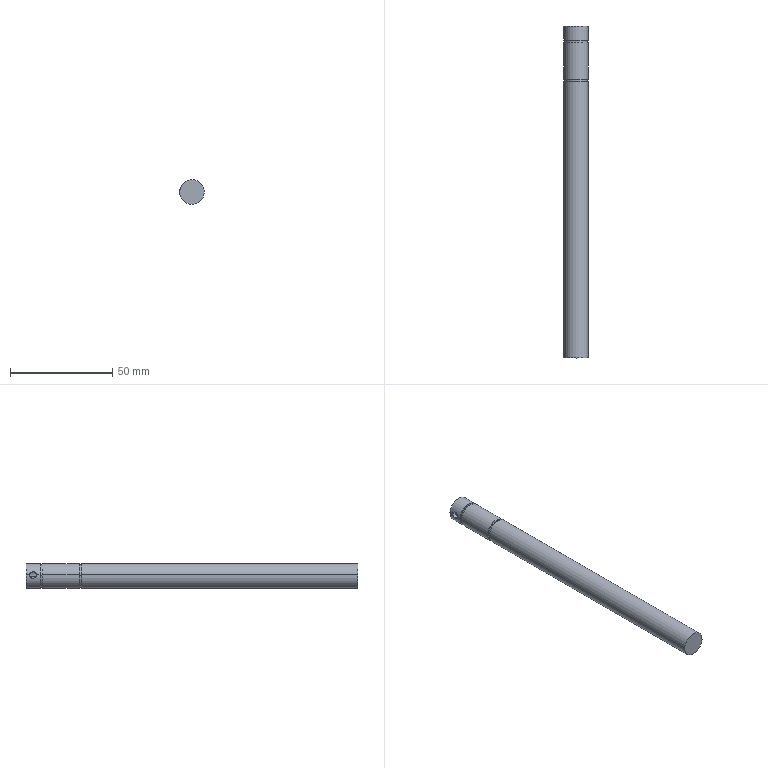Component | SolidWorks | MotorAxis-1 | 1 solid | 21 faces | box 12 x 162 x 12 mm | volume 16498 mm3 | cylinder 14 | plane 7 | commonest cylinder face diameters 12 x6 10.8 x4 3.3 x2 8 x2
build123d program:
from build123d import *

# Parameters (mm, degrees)
SKETCH1_R              = 6
BOSS_EXTRUDE1_DEPTH    = 162
SKETCH2_R              = 4
CUT_EXTRUDE1_DEPTH     = 35
SKETCH3_W              = 4.532
SKETCH3_H              = 1.1
SKETCH3_W_2            = 5.035
M4_TAPPED_HOLE1_REACH  = 161.164
M4_TAPPED_HOLE1_BORE_R = 1.65


with BuildPart() as part:
    # Sketch1 → Boss-Extrude1 (new body)
    with BuildSketch(Plane.XY):
        Circle(SKETCH1_R)
    extrude(amount=BOSS_EXTRUDE1_DEPTH)

    # Sketch2 → Cut-Extrude1 (cut)
    with BuildSketch(Plane(origin=(0, 0, 0), x_dir=(-1, 0, 0), z_dir=(0, 0, -1))):
        Circle(SKETCH2_R)
    extrude(amount=-CUT_EXTRUDE1_DEPTH, mode=Mode.SUBTRACT)

    # Sketch3 → Cut-Revolve1 (revolve, cut)
    with BuildSketch(Plane(origin=(0, 0, 0), x_dir=(1, 0, 0), z_dir=(0, 1, 0)), mode=Mode.PRIVATE) as cut_revolve1_sk:
        with Locations((7.666, -7.45)):
            Rectangle(SKETCH3_W, SKETCH3_H)
        with Locations((7.918, -26.55)):
            Rectangle(SKETCH3_W_2, SKETCH3_H)
    revolve(cut_revolve1_sk.sketch.rotate(Axis((0, 0, 0), (0, 0, 1)), 180), axis=Axis((0, 0, 0), (0, 0, 1)), mode=Mode.SUBTRACT)

    # M4 Tapped Hole1 bore (on position points) → M4 Tapped Hole1 (cut, up to next)
    with BuildSketch(Plane(origin=(-6, 0, 3.403), x_dir=(0, 0, -1), z_dir=(-1, 0, 0)), mode=Mode.PRIVATE) as m4_tapped_hole1_sk1:
        Circle(M4_TAPPED_HOLE1_BORE_R)
    m4_tapped_hole1_tool1 = extrude(m4_tapped_hole1_sk1.sketch, amount=-M4_TAPPED_HOLE1_REACH, mode=Mode.PRIVATE) & part.part
    add(m4_tapped_hole1_tool1.solids().sort_by_distance((-6, 0, 3.403))[0], mode=Mode.SUBTRACT)


solid = part.part

# Placed as in the assembly
solid = solid.moved(Location((-48.547, 4.46, 328), (90, 0, -5.004)))
STEP:
#1=COLOUR_RGB('',0.7922,0.8196,0.9333);
#2=FILL_AREA_STYLE_COLOUR('',#1);
#3=FILL_AREA_STYLE('',(#2));
#4=SURFACE_STYLE_FILL_AREA(#3);
#5=SURFACE_SIDE_STYLE('',(#4));
#6=SURFACE_STYLE_USAGE(.BOTH.,#5);
#7=PRESENTATION_STYLE_ASSIGNMENT((#6));
#8=CARTESIAN_POINT('',(-2.068,0.1066,12.927));
#9=VERTEX_POINT('',#8);
#10=CARTESIAN_POINT('',(-2.068,-0.02332,12.927));
#11=VERTEX_POINT('',#10);
#12=CARTESIAN_POINT('',(-2.068,0.1066,12.927));
#13=CARTESIAN_POINT('',(-2.069,0.1066,12.923));
#14=CARTESIAN_POINT('',(-2.069,0.1062,12.919));
#15=CARTESIAN_POINT('',(-2.069,0.1045,12.91));
#16=CARTESIAN_POINT('',(-2.069,0.1032,12.906));
#17=CARTESIAN_POINT('',(-2.068,0.0983,12.894));
#18=CARTESIAN_POINT('',(-2.067,0.09352,12.887));
#19=CARTESIAN_POINT('',(-2.065,0.08454,12.878));
#20=CARTESIAN_POINT('',(-2.064,0.0813,12.875));
#21=CARTESIAN_POINT('',(-2.063,0.07433,12.87));
#22=CARTESIAN_POINT('',(-2.062,0.07055,12.868));
#23=CARTESIAN_POINT('',(-2.061,0.06272,12.865));
#24=CARTESIAN_POINT('',(-2.061,0.05867,12.863));
#25=CARTESIAN_POINT('',(-2.06,0.05029,12.862));
#26=CARTESIAN_POINT('',(-2.06,0.04593,12.861));
#27=CARTESIAN_POINT('',(-2.06,0.03309,12.861));
#28=CARTESIAN_POINT('',(-2.061,0.02447,12.863));
#29=CARTESIAN_POINT('',(-2.062,0.01273,12.868));
#30=CARTESIAN_POINT('',(-2.063,0.008947,12.87));
#31=CARTESIAN_POINT('',(-2.064,0.001949,12.875));
#32=CARTESIAN_POINT('',(-2.065,-0.001288,12.878));
#33=CARTESIAN_POINT('',(-2.066,-0.007255,12.884));
#34=CARTESIAN_POINT('',(-2.067,-0.009956,12.887));
#35=CARTESIAN_POINT('',(-2.068,-0.01464,12.894));
#36=CARTESIAN_POINT('',(-2.068,-0.01664,12.898));
#37=CARTESIAN_POINT('',(-2.069,-0.02161,12.91));
#38=CARTESIAN_POINT('',(-2.069,-0.02332,12.918));
#39=CARTESIAN_POINT('',(-2.068,-0.02332,12.927));
#40=B_SPLINE_CURVE_WITH_KNOTS('',3,(#12,#13,#14,#15,#16,#17,#18,#19,#20,#21,#22,#23,#24,#25,#26,#27,#28,#29,#30,#31,#32,#33,#34,#35,#36,#37,#38,#39),.UNSPECIFIED.,.F.,.F.,(4,2,2,2,2,2,2,2,2,2,2,2,2,4),(0.005218,0.005543,0.005869,0.006521,0.006847,0.007173,0.007499,0.007824,0.008476,0.008802,0.009128,0.009454,0.009779,0.01043),.UNSPECIFIED.);
#41=EDGE_CURVE('',#9,#11,#40,.T.);
#42=ORIENTED_EDGE('',*,*,#41,.F.);
#43=CARTESIAN_POINT('',(-2.147,0.1066,12.934));
#44=VERTEX_POINT('',#43);
#45=CARTESIAN_POINT('',(-2.147,0.1066,12.934));
#46=DIRECTION('',(-0.9962,-0.,0.08723));
#47=VECTOR('',#46,39.37);
#48=LINE('',#45,#47);
#49=EDGE_CURVE('',#9,#44,#48,.T.);
#50=ORIENTED_EDGE('',*,*,#49,.T.);
#51=CARTESIAN_POINT('',(-2.147,-0.02332,12.934));
#52=VERTEX_POINT('',#51);
#53=CARTESIAN_POINT('',(-2.147,-0.02332,12.934));
#54=CARTESIAN_POINT('',(-2.147,-0.02332,12.93));
#55=CARTESIAN_POINT('',(-2.147,-0.0229,12.925));
#56=CARTESIAN_POINT('',(-2.148,-0.02123,12.917));
#57=CARTESIAN_POINT('',(-2.148,-0.01997,12.913));
#58=CARTESIAN_POINT('',(-2.147,-0.0167,12.905));
#59=CARTESIAN_POINT('',(-2.147,-0.01471,12.901));
#60=CARTESIAN_POINT('',(-2.147,-0.009991,12.894));
#61=CARTESIAN_POINT('',(-2.146,-0.007262,12.891));
#62=CARTESIAN_POINT('',(-2.145,0.001683,12.882));
#63=CARTESIAN_POINT('',(-2.145,0.008896,12.877));
#64=CARTESIAN_POINT('',(-2.144,0.02451,12.87));
#65=CARTESIAN_POINT('',(-2.143,0.03309,12.868));
#66=CARTESIAN_POINT('',(-2.143,0.04587,12.868));
#67=CARTESIAN_POINT('',(-2.143,0.0502,12.869));
#68=CARTESIAN_POINT('',(-2.144,0.05855,12.871));
#69=CARTESIAN_POINT('',(-2.144,0.06261,12.872));
#70=CARTESIAN_POINT('',(-2.145,0.07444,12.877));
#71=CARTESIAN_POINT('',(-2.145,0.08158,12.882));
#72=CARTESIAN_POINT('',(-2.146,0.09059,12.891));
#73=CARTESIAN_POINT('',(-2.147,0.09326,12.894));
#74=CARTESIAN_POINT('',(-2.147,0.09796,12.901));
#75=CARTESIAN_POINT('',(-2.147,0.1,12.905));
#76=CARTESIAN_POINT('',(-2.148,0.1033,12.913));
#77=CARTESIAN_POINT('',(-2.148,0.1045,12.917));
#78=CARTESIAN_POINT('',(-2.147,0.1062,12.925));
#79=CARTESIAN_POINT('',(-2.147,0.1066,12.93));
#80=CARTESIAN_POINT('',(-2.147,0.1066,12.934));
#81=B_SPLINE_CURVE_WITH_KNOTS('',3,(#53,#54,#55,#56,#57,#58,#59,#60,#61,#62,#63,#64,#65,#66,#67,#68,#69,#70,#71,#72,#73,#74,#75,#76,#77,#78,#79,#80),.UNSPECIFIED.,.F.,.F.,(4,2,2,2,2,2,2,2,2,2,2,2,2,4),(0.,0.000324,0.000648,0.000972,0.001296,0.001944,0.002592,0.002916,0.00324,0.003888,0.004212,0.004536,0.00486,0.005184),.UNSPECIFIED.);
#82=EDGE_CURVE('',#52,#44,#81,.T.);
#83=ORIENTED_EDGE('',*,*,#82,.F.);
#84=CARTESIAN_POINT('',(-2.147,-0.02332,12.934));
#85=DIRECTION('',(-0.9962,-0.,0.08723));
#86=VECTOR('',#85,39.37);
#87=LINE('',#84,#86);
#88=EDGE_CURVE('',#11,#52,#87,.T.);
#89=ORIENTED_EDGE('',*,*,#88,.F.);
#90=EDGE_LOOP('',(#42,#50,#83,#89));
#91=FACE_OUTER_BOUND('',#90,.T.);
#92=CARTESIAN_POINT('',(-2.147,0.04164,12.934));
#93=DIRECTION('',(-0.9962,-0.,0.08723));
#94=DIRECTION('',(0.,-1.,0.));
#95=AXIS2_PLACEMENT_3D('',#92,#93,#94);
#96=CYLINDRICAL_SURFACE('',#95,0.06496);
#97=ADVANCED_FACE('',(#91),#96,.F.);
#98=CARTESIAN_POINT('',(-1.676,-6.202,12.893));
#99=VERTEX_POINT('',#98);
#100=CARTESIAN_POINT('',(-2.147,-6.202,12.934));
#101=VERTEX_POINT('',#100);
#102=CARTESIAN_POINT('',(-1.911,-6.202,12.913));
#103=DIRECTION('',(0.,-1.,0.));
#104=DIRECTION('',(0.9962,0.,-0.08723));
#105=AXIS2_PLACEMENT_3D('',#102,#103,#104);
#106=CIRCLE('',#105,0.2362);
#107=EDGE_CURVE('',#99,#101,#106,.T.);
#108=ORIENTED_EDGE('',*,*,#107,.F.);
#109=CARTESIAN_POINT('',(-1.676,-0.8913,12.893));
#110=VERTEX_POINT('',#109);
#111=CARTESIAN_POINT('',(-1.676,-6.202,12.893));
#112=DIRECTION('',(-0.,1.,-0.));
#113=VECTOR('',#112,39.37);
#114=LINE('',#111,#113);
#115=EDGE_CURVE('',#99,#110,#114,.T.);
#116=ORIENTED_EDGE('',*,*,#115,.T.);
#117=CARTESIAN_POINT('',(-2.147,-0.8913,12.934));
#118=VERTEX_POINT('',#117);
#119=CARTESIAN_POINT('',(-1.911,-0.8913,12.913));
#120=DIRECTION('',(-0.,1.,-0.));
#121=DIRECTION('',(-0.9962,-0.,0.08723));
#122=AXIS2_PLACEMENT_3D('',#119,#120,#121);
#123=CIRCLE('',#122,0.2362);
#124=EDGE_CURVE('',#118,#110,#123,.T.);
#125=ORIENTED_EDGE('',*,*,#124,.F.);
#126=CARTESIAN_POINT('',(-2.147,-6.202,12.934));
#127=DIRECTION('',(-0.,1.,-0.));
#128=VECTOR('',#127,39.37);
#129=LINE('',#126,#128);
#130=EDGE_CURVE('',#101,#118,#129,.T.);
#131=ORIENTED_EDGE('',*,*,#130,.F.);
#132=EDGE_LOOP('',(#108,#116,#125,#131));
#133=FACE_OUTER_BOUND('',#132,.T.);
#134=CARTESIAN_POINT('',(-1.911,-6.202,12.913));
#135=DIRECTION('',(-0.,1.,-0.));
#136=DIRECTION('',(-0.9962,0.,0.08723));
#137=AXIS2_PLACEMENT_3D('',#134,#135,#136);
#138=CYLINDRICAL_SURFACE('',#137,0.2362);
#139=ADVANCED_FACE('',(#133),#138,.T.);
#140=CARTESIAN_POINT('',(-2.123,-0.8913,12.932));
#141=VERTEX_POINT('',#140);
#142=CARTESIAN_POINT('',(-1.7,-0.8913,12.895));
#143=VERTEX_POINT('',#142);
#144=CARTESIAN_POINT('',(-1.911,-0.8913,12.913));
#145=DIRECTION('',(-0.,1.,-0.));
#146=DIRECTION('',(-0.9962,-0.,0.08723));
#147=AXIS2_PLACEMENT_3D('',#144,#145,#146);
#148=CIRCLE('',#147,0.2126);
#149=EDGE_CURVE('',#141,#143,#148,.T.);
#150=ORIENTED_EDGE('',*,*,#149,.T.);
#151=CARTESIAN_POINT('',(-1.7,-0.848,12.895));
#152=VERTEX_POINT('',#151);
#153=CARTESIAN_POINT('',(-1.7,0.1756,12.895));
#154=DIRECTION('',(-0.,1.,-0.));
#155=VECTOR('',#154,39.37);
#156=LINE('',#153,#155);
#157=EDGE_CURVE('',#143,#152,#156,.T.);
#158=ORIENTED_EDGE('',*,*,#157,.T.);
#159=CARTESIAN_POINT('',(-2.123,-0.848,12.932));
#160=VERTEX_POINT('',#159);
#161=CARTESIAN_POINT('',(-1.911,-0.848,12.913));
#162=DIRECTION('',(-0.,1.,-0.));
#163=DIRECTION('',(-0.9962,-0.,0.08723));
#164=AXIS2_PLACEMENT_3D('',#161,#162,#163);
#165=CIRCLE('',#164,0.2126);
#166=EDGE_CURVE('',#160,#152,#165,.T.);
#167=ORIENTED_EDGE('',*,*,#166,.F.);
#168=CARTESIAN_POINT('',(-2.123,0.1756,12.932));
#169=DIRECTION('',(-0.,1.,-0.));
#170=VECTOR('',#169,39.37);
#171=LINE('',#168,#170);
#172=EDGE_CURVE('',#141,#160,#171,.T.);
#173=ORIENTED_EDGE('',*,*,#172,.F.);
#174=EDGE_LOOP('',(#150,#158,#167,#173));
#175=FACE_OUTER_BOUND('',#174,.T.);
#176=CARTESIAN_POINT('',(-1.911,0.1756,12.913));
#177=DIRECTION('',(-0.,1.,-0.));
#178=DIRECTION('',(-0.9962,-0.,0.08723));
#179=AXIS2_PLACEMENT_3D('',#176,#177,#178);
#180=CYLINDRICAL_SURFACE('',#179,0.2126);
#181=ADVANCED_FACE('',(#175),#180,.T.);
#182=CARTESIAN_POINT('',(-2.123,-0.1394,12.932));
#183=VERTEX_POINT('',#182);
#184=CARTESIAN_POINT('',(-1.7,-0.1394,12.895));
#185=VERTEX_POINT('',#184);
#186=CARTESIAN_POINT('',(-1.911,-0.1394,12.913));
#187=DIRECTION('',(-0.,1.,-0.));
#188=DIRECTION('',(-0.9962,-0.,0.08723));
#189=AXIS2_PLACEMENT_3D('',#186,#187,#188);
#190=CIRCLE('',#189,0.2126);
#191=EDGE_CURVE('',#183,#185,#190,.T.);
#192=ORIENTED_EDGE('',*,*,#191,.T.);
#193=CARTESIAN_POINT('',(-1.7,-0.09605,12.895));
#194=VERTEX_POINT('',#193);
#195=CARTESIAN_POINT('',(-1.7,0.1756,12.895));
#196=DIRECTION('',(-0.,1.,-0.));
#197=VECTOR('',#196,39.37);
#198=LINE('',#195,#197);
#199=EDGE_CURVE('',#185,#194,#198,.T.);
#200=ORIENTED_EDGE('',*,*,#199,.T.);
#201=CARTESIAN_POINT('',(-2.123,-0.09605,12.932));
#202=VERTEX_POINT('',#201);
#203=CARTESIAN_POINT('',(-1.911,-0.09605,12.913));
#204=DIRECTION('',(-0.,1.,-0.));
#205=DIRECTION('',(-0.9962,-0.,0.08723));
#206=AXIS2_PLACEMENT_3D('',#203,#204,#205);
#207=CIRCLE('',#206,0.2126);
#208=EDGE_CURVE('',#202,#194,#207,.T.);
#209=ORIENTED_EDGE('',*,*,#208,.F.);
#210=CARTESIAN_POINT('',(-2.123,0.1756,12.932));
#211=DIRECTION('',(-0.,1.,-0.));
#212=VECTOR('',#211,39.37);
#213=LINE('',#210,#212);
#214=EDGE_CURVE('',#183,#202,#213,.T.);
#215=ORIENTED_EDGE('',*,*,#214,.F.);
#216=EDGE_LOOP('',(#192,#200,#209,#215));
#217=FACE_OUTER_BOUND('',#216,.T.);
#218=CARTESIAN_POINT('',(-1.911,0.1756,12.913));
#219=DIRECTION('',(-0.,1.,-0.));
#220=DIRECTION('',(-0.9962,-0.,0.08723));
#221=AXIS2_PLACEMENT_3D('',#218,#219,#220);
#222=CYLINDRICAL_SURFACE('',#221,0.2126);
#223=ADVANCED_FACE('',(#217),#222,.T.);
#224=CARTESIAN_POINT('',(-1.754,-1.202,12.9));
#225=VERTEX_POINT('',#224);
#226=CARTESIAN_POINT('',(-2.068,-1.202,12.927));
#227=VERTEX_POINT('',#226);
#228=CARTESIAN_POINT('',(-1.911,-1.202,12.913));
#229=DIRECTION('',(-0.,1.,-0.));
#230=DIRECTION('',(-0.9962,-0.,0.08723));
#231=AXIS2_PLACEMENT_3D('',#228,#229,#230);
#232=CIRCLE('',#231,0.1575);
#233=EDGE_CURVE('',#225,#227,#232,.T.);
#234=ORIENTED_EDGE('',*,*,#233,.F.);
#235=CARTESIAN_POINT('',(-1.754,0.1756,12.9));
#236=VERTEX_POINT('',#235);
#237=CARTESIAN_POINT('',(-1.754,-1.202,12.9));
#238=DIRECTION('',(-0.,1.,-0.));
#239=VECTOR('',#238,39.37);
#240=LINE('',#237,#239);
#241=EDGE_CURVE('',#225,#236,#240,.T.);
#242=ORIENTED_EDGE('',*,*,#241,.T.);
#243=CARTESIAN_POINT('',(-2.068,0.1756,12.927));
#244=VERTEX_POINT('',#243);
#245=CARTESIAN_POINT('',(-1.911,0.1756,12.913));
#246=DIRECTION('',(-0.,1.,-0.));
#247=DIRECTION('',(-0.9962,-0.,0.08723));
#248=AXIS2_PLACEMENT_3D('',#245,#246,#247);
#249=CIRCLE('',#248,0.1575);
#250=EDGE_CURVE('',#236,#244,#249,.T.);
#251=ORIENTED_EDGE('',*,*,#250,.T.);
#252=CARTESIAN_POINT('',(-2.068,-1.202,12.927));
#253=DIRECTION('',(-0.,1.,-0.));
#254=VECTOR('',#253,39.37);
#255=LINE('',#252,#254);
#256=EDGE_CURVE('',#9,#244,#255,.T.);
#257=ORIENTED_EDGE('',*,*,#256,.F.);
#258=ORIENTED_EDGE('',*,*,#41,.T.);
#259=CARTESIAN_POINT('',(-2.068,-1.202,12.927));
#260=DIRECTION('',(-0.,1.,-0.));
#261=VECTOR('',#260,39.37);
#262=LINE('',#259,#261);
#263=EDGE_CURVE('',#227,#11,#262,.T.);
#264=ORIENTED_EDGE('',*,*,#263,.F.);
#265=EDGE_LOOP('',(#234,#242,#251,#257,#258,#264));
#266=FACE_OUTER_BOUND('',#265,.T.);
#267=CARTESIAN_POINT('',(-1.911,-1.202,12.913));
#268=DIRECTION('',(-0.,1.,-0.));
#269=DIRECTION('',(-0.9962,-0.,0.08723));
#270=AXIS2_PLACEMENT_3D('',#267,#268,#269);
#271=CYLINDRICAL_SURFACE('',#270,0.1575);
#272=ADVANCED_FACE('',(#266),#271,.F.);
#273=CARTESIAN_POINT('',(-1.676,-0.09605,12.893));
#274=VERTEX_POINT('',#273);
#275=CARTESIAN_POINT('',(-2.147,-0.09605,12.934));
#276=VERTEX_POINT('',#275);
#277=CARTESIAN_POINT('',(-1.911,-0.09605,12.913));
#278=DIRECTION('',(0.,-1.,0.));
#279=DIRECTION('',(0.9962,0.,-0.08723));
#280=AXIS2_PLACEMENT_3D('',#277,#278,#279);
#281=CIRCLE('',#280,0.2362);
#282=EDGE_CURVE('',#274,#276,#281,.T.);
#283=ORIENTED_EDGE('',*,*,#282,.F.);
#284=CARTESIAN_POINT('',(-1.676,0.1756,12.893));
#285=VERTEX_POINT('',#284);
#286=CARTESIAN_POINT('',(-1.676,-6.202,12.893));
#287=DIRECTION('',(-0.,1.,-0.));
#288=VECTOR('',#287,39.37);
#289=LINE('',#286,#288);
#290=EDGE_CURVE('',#274,#285,#289,.T.);
#291=ORIENTED_EDGE('',*,*,#290,.T.);
#292=CARTESIAN_POINT('',(-2.147,0.1756,12.934));
#293=VERTEX_POINT('',#292);
#294=CARTESIAN_POINT('',(-1.911,0.1756,12.913));
#295=DIRECTION('',(0.,-1.,0.));
#296=DIRECTION('',(0.9962,0.,-0.08723));
#297=AXIS2_PLACEMENT_3D('',#294,#295,#296);
#298=CIRCLE('',#297,0.2362);
#299=EDGE_CURVE('',#285,#293,#298,.T.);
#300=ORIENTED_EDGE('',*,*,#299,.T.);
#301=CARTESIAN_POINT('',(-2.147,-6.202,12.934));
#302=DIRECTION('',(-0.,1.,-0.));
#303=VECTOR('',#302,39.37);
#304=LINE('',#301,#303);
#305=EDGE_CURVE('',#44,#293,#304,.T.);
#306=ORIENTED_EDGE('',*,*,#305,.F.);
#307=CARTESIAN_POINT('',(-2.147,0.1066,12.934));
#308=CARTESIAN_POINT('',(-2.146,0.1066,12.942));
#309=CARTESIAN_POINT('',(-2.145,0.1049,12.951));
#310=CARTESIAN_POINT('',(-2.142,0.1,12.963));
#311=CARTESIAN_POINT('',(-2.142,0.09797,12.966));
#312=CARTESIAN_POINT('',(-2.14,0.09325,12.973));
#313=CARTESIAN_POINT('',(-2.139,0.09058,12.976));
#314=CARTESIAN_POINT('',(-2.137,0.08459,12.982));
#315=CARTESIAN_POINT('',(-2.136,0.08127,12.985));
#316=CARTESIAN_POINT('',(-2.135,0.07427,12.99));
#317=CARTESIAN_POINT('',(-2.134,0.07054,12.991));
#318=CARTESIAN_POINT('',(-2.133,0.06263,12.995));
#319=CARTESIAN_POINT('',(-2.133,0.05856,12.996));
#320=CARTESIAN_POINT('',(-2.132,0.05024,12.997));
#321=CARTESIAN_POINT('',(-2.132,0.04593,12.998));
#322=CARTESIAN_POINT('',(-2.132,0.03737,12.998));
#323=CARTESIAN_POINT('',(-2.132,0.03314,12.998));
#324=CARTESIAN_POINT('',(-2.133,0.02478,12.996));
#325=CARTESIAN_POINT('',(-2.133,0.02064,12.995));
#326=CARTESIAN_POINT('',(-2.135,0.008894,12.99));
#327=CARTESIAN_POINT('',(-2.136,0.001688,12.985));
#328=CARTESIAN_POINT('',(-2.14,-0.01023,12.974));
#329=CARTESIAN_POINT('',(-2.142,-0.01507,12.966));
#330=CARTESIAN_POINT('',(-2.144,-0.01996,12.955));
#331=CARTESIAN_POINT('',(-2.145,-0.02122,12.951));
#332=CARTESIAN_POINT('',(-2.146,-0.0229,12.943));
#333=CARTESIAN_POINT('',(-2.146,-0.02332,12.938));
#334=CARTESIAN_POINT('',(-2.147,-0.02332,12.934));
#335=B_SPLINE_CURVE_WITH_KNOTS('',3,(#307,#308,#309,#310,#311,#312,#313,#314,#315,#316,#317,#318,#319,#320,#321,#322,#323,#324,#325,#326,#327,#328,#329,#330,#331,#332,#333,#334),.UNSPECIFIED.,.F.,.F.,(4,2,2,2,2,2,2,2,2,2,2,2,2,4),(0.005184,0.005832,0.006155,0.006479,0.006803,0.007127,0.007451,0.007775,0.008099,0.008423,0.00907,0.009718,0.01004,0.01037),.UNSPECIFIED.);
#336=EDGE_CURVE('',#44,#52,#335,.T.);
#337=ORIENTED_EDGE('',*,*,#336,.T.);
#338=CARTESIAN_POINT('',(-2.147,-6.202,12.934));
#339=DIRECTION('',(-0.,1.,-0.));
#340=VECTOR('',#339,39.37);
#341=LINE('',#338,#340);
#342=EDGE_CURVE('',#276,#52,#341,.T.);
#343=ORIENTED_EDGE('',*,*,#342,.F.);
#344=EDGE_LOOP('',(#283,#291,#300,#306,#337,#343));
#345=FACE_OUTER_BOUND('',#344,.T.);
#346=CARTESIAN_POINT('',(-1.911,-6.202,12.913));
#347=DIRECTION('',(-0.,1.,-0.));
#348=DIRECTION('',(-0.9962,0.,0.08723));
#349=AXIS2_PLACEMENT_3D('',#346,#347,#348);
#350=CYLINDRICAL_SURFACE('',#349,0.2362);
#351=ADVANCED_FACE('',(#345),#350,.T.);
#352=CARTESIAN_POINT('',(-1.676,-0.848,12.893));
#353=VERTEX_POINT('',#352);
#354=CARTESIAN_POINT('',(-2.147,-0.848,12.934));
#355=VERTEX_POINT('',#354);
#356=CARTESIAN_POINT('',(-1.911,-0.848,12.913));
#357=DIRECTION('',(0.,-1.,0.));
#358=DIRECTION('',(0.9962,0.,-0.08723));
#359=AXIS2_PLACEMENT_3D('',#356,#357,#358);
#360=CIRCLE('',#359,0.2362);
#361=EDGE_CURVE('',#353,#355,#360,.T.);
#362=ORIENTED_EDGE('',*,*,#361,.F.);
#363=CARTESIAN_POINT('',(-1.676,-0.1394,12.893));
#364=VERTEX_POINT('',#363);
#365=CARTESIAN_POINT('',(-1.676,-6.202,12.893));
#366=DIRECTION('',(-0.,1.,-0.));
#367=VECTOR('',#366,39.37);
#368=LINE('',#365,#367);
#369=EDGE_CURVE('',#353,#364,#368,.T.);
#370=ORIENTED_EDGE('',*,*,#369,.T.);
#371=CARTESIAN_POINT('',(-2.147,-0.1394,12.934));
#372=VERTEX_POINT('',#371);
#373=CARTESIAN_POINT('',(-1.911,-0.1394,12.913));
#374=DIRECTION('',(-0.,1.,-0.));
#375=DIRECTION('',(-0.9962,-0.,0.08723));
#376=AXIS2_PLACEMENT_3D('',#373,#374,#375);
#377=CIRCLE('',#376,0.2362);
#378=EDGE_CURVE('',#372,#364,#377,.T.);
#379=ORIENTED_EDGE('',*,*,#378,.F.);
#380=CARTESIAN_POINT('',(-2.147,-6.202,12.934));
#381=DIRECTION('',(-0.,1.,-0.));
#382=VECTOR('',#381,39.37);
#383=LINE('',#380,#382);
#384=EDGE_CURVE('',#355,#372,#383,.T.);
#385=ORIENTED_EDGE('',*,*,#384,.F.);
#386=EDGE_LOOP('',(#362,#370,#379,#385));
#387=FACE_OUTER_BOUND('',#386,.T.);
#388=CARTESIAN_POINT('',(-1.911,-6.202,12.913));
#389=DIRECTION('',(-0.,1.,-0.));
#390=DIRECTION('',(-0.9962,0.,0.08723));
#391=AXIS2_PLACEMENT_3D('',#388,#389,#390);
#392=CYLINDRICAL_SURFACE('',#391,0.2362);
#393=ADVANCED_FACE('',(#387),#392,.T.);
#394=ORIENTED_EDGE('',*,*,#369,.F.);
#395=CARTESIAN_POINT('',(-1.911,-0.848,12.913));
#396=DIRECTION('',(0.,-1.,0.));
#397=DIRECTION('',(0.9962,0.,-0.08723));
#398=AXIS2_PLACEMENT_3D('',#395,#396,#397);
#399=CIRCLE('',#398,0.2362);
#400=EDGE_CURVE('',#355,#353,#399,.T.);
#401=ORIENTED_EDGE('',*,*,#400,.F.);
#402=ORIENTED_EDGE('',*,*,#384,.T.);
#403=CARTESIAN_POINT('',(-1.911,-0.1394,12.913));
#404=DIRECTION('',(-0.,1.,-0.));
#405=DIRECTION('',(-0.9962,-0.,0.08723));
#406=AXIS2_PLACEMENT_3D('',#403,#404,#405);
#407=CIRCLE('',#406,0.2362);
#408=EDGE_CURVE('',#364,#372,#407,.T.);
#409=ORIENTED_EDGE('',*,*,#408,.F.);
#410=EDGE_LOOP('',(#394,#401,#402,#409));
#411=FACE_OUTER_BOUND('',#410,.T.);
#412=CARTESIAN_POINT('',(-1.911,-6.202,12.913));
#413=DIRECTION('',(-0.,1.,-0.));
#414=DIRECTION('',(-0.9962,0.,0.08723));
#415=AXIS2_PLACEMENT_3D('',#412,#413,#414);
#416=CYLINDRICAL_SURFACE('',#415,0.2362);
#417=ADVANCED_FACE('',(#411),#416,.T.);
#418=ORIENTED_EDGE('',*,*,#290,.F.);
#419=CARTESIAN_POINT('',(-1.911,-0.09605,12.913));
#420=DIRECTION('',(0.,-1.,0.));
#421=DIRECTION('',(0.9962,0.,-0.08723));
#422=AXIS2_PLACEMENT_3D('',#419,#420,#421);
#423=CIRCLE('',#422,0.2362);
#424=EDGE_CURVE('',#276,#274,#423,.T.);
#425=ORIENTED_EDGE('',*,*,#424,.F.);
#426=ORIENTED_EDGE('',*,*,#342,.T.);
#427=ORIENTED_EDGE('',*,*,#82,.T.);
#428=ORIENTED_EDGE('',*,*,#305,.T.);
#429=CARTESIAN_POINT('',(-1.911,0.1756,12.913));
#430=DIRECTION('',(0.,-1.,0.));
#431=DIRECTION('',(0.9962,0.,-0.08723));
#432=AXIS2_PLACEMENT_3D('',#429,#430,#431);
#433=CIRCLE('',#432,0.2362);
#434=EDGE_CURVE('',#293,#285,#433,.T.);
#435=ORIENTED_EDGE('',*,*,#434,.T.);
#436=EDGE_LOOP('',(#418,#425,#426,#427,#428,#435));
#437=FACE_OUTER_BOUND('',#436,.T.);
#438=CARTESIAN_POINT('',(-1.911,-6.202,12.913));
#439=DIRECTION('',(-0.,1.,-0.));
#440=DIRECTION('',(-0.9962,0.,0.08723));
#441=AXIS2_PLACEMENT_3D('',#438,#439,#440);
#442=CYLINDRICAL_SURFACE('',#441,0.2362);
#443=ADVANCED_FACE('',(#437),#442,.T.);
#444=CARTESIAN_POINT('',(-1.911,0.1756,12.913));
#445=DIRECTION('',(-0.,1.,-0.));
#446=DIRECTION('',(-0.9962,-0.,0.08723));
#447=AXIS2_PLACEMENT_3D('',#444,#445,#446);
#448=CIRCLE('',#447,0.1575);
#449=EDGE_CURVE('',#244,#236,#448,.T.);
#450=ORIENTED_EDGE('',*,*,#449,.F.);
#451=ORIENTED_EDGE('',*,*,#250,.F.);
#452=EDGE_LOOP('',(#450,#451));
#453=FACE_BOUND('',#452,.T.);
#454=ORIENTED_EDGE('',*,*,#434,.F.);
#455=ORIENTED_EDGE('',*,*,#299,.F.);
#456=EDGE_LOOP('',(#454,#455));
#457=FACE_OUTER_BOUND('',#456,.T.);
#458=CARTESIAN_POINT('',(-1.911,0.1756,12.913));
#459=DIRECTION('',(0.,-1.,0.));
#460=DIRECTION('',(0.9962,0.,-0.08723));
#461=AXIS2_PLACEMENT_3D('',#458,#459,#460);
#462=PLANE('',#461);
#463=ADVANCED_FACE('',(#453,#457),#462,.F.);
#464=ORIENTED_EDGE('',*,*,#241,.F.);
#465=CARTESIAN_POINT('',(-1.911,-1.202,12.913));
#466=DIRECTION('',(-0.,1.,-0.));
#467=DIRECTION('',(-0.9962,-0.,0.08723));
#468=AXIS2_PLACEMENT_3D('',#465,#466,#467);
#469=CIRCLE('',#468,0.1575);
#470=EDGE_CURVE('',#227,#225,#469,.T.);
#471=ORIENTED_EDGE('',*,*,#470,.F.);
#472=ORIENTED_EDGE('',*,*,#263,.T.);
#473=CARTESIAN_POINT('',(-2.068,-0.02332,12.927));
#474=CARTESIAN_POINT('',(-2.068,-0.02332,12.931));
#475=CARTESIAN_POINT('',(-2.067,-0.02289,12.936));
#476=CARTESIAN_POINT('',(-2.066,-0.02121,12.944));
#477=CARTESIAN_POINT('',(-2.065,-0.01994,12.948));
#478=CARTESIAN_POINT('',(-2.062,-0.01501,12.96));
#479=CARTESIAN_POINT('',(-2.06,-0.01019,12.967));
#480=CARTESIAN_POINT('',(-2.055,0.001663,12.978));
#481=CARTESIAN_POINT('',(-2.053,0.008817,12.983));
#482=CARTESIAN_POINT('',(-2.05,0.02051,12.987));
#483=CARTESIAN_POINT('',(-2.05,0.02465,12.989));
#484=CARTESIAN_POINT('',(-2.049,0.03306,12.99));
#485=CARTESIAN_POINT('',(-2.049,0.0373,12.991));
#486=CARTESIAN_POINT('',(-2.049,0.04589,12.991));
#487=CARTESIAN_POINT('',(-2.049,0.05025,12.99));
#488=CARTESIAN_POINT('',(-2.05,0.05862,12.989));
#489=CARTESIAN_POINT('',(-2.05,0.06271,12.987));
#490=CARTESIAN_POINT('',(-2.052,0.07062,12.984));
#491=CARTESIAN_POINT('',(-2.053,0.07433,12.982));
#492=CARTESIAN_POINT('',(-2.055,0.08132,12.978));
#493=CARTESIAN_POINT('',(-2.056,0.08462,12.975));
#494=CARTESIAN_POINT('',(-2.059,0.09056,12.969));
#495=CARTESIAN_POINT('',(-2.06,0.09322,12.966));
#496=CARTESIAN_POINT('',(-2.062,0.09793,12.959));
#497=CARTESIAN_POINT('',(-2.063,0.09996,12.956));
#498=CARTESIAN_POINT('',(-2.066,0.1048,12.944));
#499=CARTESIAN_POINT('',(-2.067,0.1066,12.936));
#500=CARTESIAN_POINT('',(-2.068,0.1066,12.927));
#501=B_SPLINE_CURVE_WITH_KNOTS('',3,(#473,#474,#475,#476,#477,#478,#479,#480,#481,#482,#483,#484,#485,#486,#487,#488,#489,#490,#491,#492,#493,#494,#495,#496,#497,#498,#499,#500),.UNSPECIFIED.,.F.,.F.,(4,2,2,2,2,2,2,2,2,2,2,2,2,4),(0.,0.0003261,0.0006522,0.001304,0.001957,0.002283,0.002609,0.002935,0.003261,0.003587,0.003913,0.004239,0.004565,0.005218),.UNSPECIFIED.);
#502=EDGE_CURVE('',#11,#9,#501,.T.);
#503=ORIENTED_EDGE('',*,*,#502,.T.);
#504=ORIENTED_EDGE('',*,*,#256,.T.);
#505=ORIENTED_EDGE('',*,*,#449,.T.);
#506=EDGE_LOOP('',(#464,#471,#472,#503,#504,#505));
#507=FACE_OUTER_BOUND('',#506,.T.);
#508=CARTESIAN_POINT('',(-1.911,-1.202,12.913));
#509=DIRECTION('',(-0.,1.,-0.));
#510=DIRECTION('',(-0.9962,-0.,0.08723));
#511=AXIS2_PLACEMENT_3D('',#508,#509,#510);
#512=CYLINDRICAL_SURFACE('',#511,0.1575);
#513=ADVANCED_FACE('',(#507),#512,.F.);
#514=ORIENTED_EDGE('',*,*,#470,.T.);
#515=ORIENTED_EDGE('',*,*,#233,.T.);
#516=EDGE_LOOP('',(#514,#515));
#517=FACE_OUTER_BOUND('',#516,.T.);
#518=CARTESIAN_POINT('',(-1.911,-1.202,12.913));
#519=DIRECTION('',(-0.,1.,-0.));
#520=DIRECTION('',(-0.9962,-0.,0.08723));
#521=AXIS2_PLACEMENT_3D('',#518,#519,#520);
#522=PLANE('',#521);
#523=ADVANCED_FACE('',(#517),#522,.T.);
#524=ORIENTED_EDGE('',*,*,#191,.F.);
#525=CARTESIAN_POINT('',(-1.911,-0.1394,12.913));
#526=DIRECTION('',(-0.,1.,-0.));
#527=DIRECTION('',(-0.9962,-0.,0.08723));
#528=AXIS2_PLACEMENT_3D('',#525,#526,#527);
#529=CIRCLE('',#528,0.2126);
#530=EDGE_CURVE('',#185,#183,#529,.T.);
#531=ORIENTED_EDGE('',*,*,#530,.F.);
#532=EDGE_LOOP('',(#524,#531));
#533=FACE_BOUND('',#532,.T.);
#534=ORIENTED_EDGE('',*,*,#378,.T.);
#535=ORIENTED_EDGE('',*,*,#408,.T.);
#536=EDGE_LOOP('',(#534,#535));
#537=FACE_OUTER_BOUND('',#536,.T.);
#538=CARTESIAN_POINT('',(-1.7,-0.1394,12.895));
#539=DIRECTION('',(-0.,1.,-0.));
#540=DIRECTION('',(-0.9962,-0.,0.08723));
#541=AXIS2_PLACEMENT_3D('',#538,#539,#540);
#542=PLANE('',#541);
#543=ADVANCED_FACE('',(#533,#537),#542,.T.);
#544=ORIENTED_EDGE('',*,*,#208,.T.);
#545=CARTESIAN_POINT('',(-1.911,-0.09605,12.913));
#546=DIRECTION('',(-0.,1.,-0.));
#547=DIRECTION('',(-0.9962,-0.,0.08723));
#548=AXIS2_PLACEMENT_3D('',#545,#546,#547);
#549=CIRCLE('',#548,0.2126);
#550=EDGE_CURVE('',#194,#202,#549,.T.);
#551=ORIENTED_EDGE('',*,*,#550,.T.);
#552=EDGE_LOOP('',(#544,#551));
#553=FACE_BOUND('',#552,.T.);
#554=ORIENTED_EDGE('',*,*,#424,.T.);
#555=ORIENTED_EDGE('',*,*,#282,.T.);
#556=EDGE_LOOP('',(#554,#555));
#557=FACE_OUTER_BOUND('',#556,.T.);
#558=CARTESIAN_POINT('',(-1.7,-0.09605,12.895));
#559=DIRECTION('',(0.,-1.,0.));
#560=DIRECTION('',(0.9962,0.,-0.08723));
#561=AXIS2_PLACEMENT_3D('',#558,#559,#560);
#562=PLANE('',#561);
#563=ADVANCED_FACE('',(#553,#557),#562,.T.);
#564=ORIENTED_EDGE('',*,*,#199,.F.);
#565=ORIENTED_EDGE('',*,*,#530,.T.);
#566=ORIENTED_EDGE('',*,*,#214,.T.);
#567=ORIENTED_EDGE('',*,*,#550,.F.);
#568=EDGE_LOOP('',(#564,#565,#566,#567));
#569=FACE_OUTER_BOUND('',#568,.T.);
#570=CARTESIAN_POINT('',(-1.911,0.1756,12.913));
#571=DIRECTION('',(-0.,1.,-0.));
#572=DIRECTION('',(-0.9962,-0.,0.08723));
#573=AXIS2_PLACEMENT_3D('',#570,#571,#572);
#574=CYLINDRICAL_SURFACE('',#573,0.2126);
#575=ADVANCED_FACE('',(#569),#574,.T.);
#576=ORIENTED_EDGE('',*,*,#149,.F.);
#577=CARTESIAN_POINT('',(-1.911,-0.8913,12.913));
#578=DIRECTION('',(-0.,1.,-0.));
#579=DIRECTION('',(-0.9962,-0.,0.08723));
#580=AXIS2_PLACEMENT_3D('',#577,#578,#579);
#581=CIRCLE('',#580,0.2126);
#582=EDGE_CURVE('',#143,#141,#581,.T.);
#583=ORIENTED_EDGE('',*,*,#582,.F.);
#584=EDGE_LOOP('',(#576,#583));
#585=FACE_BOUND('',#584,.T.);
#586=ORIENTED_EDGE('',*,*,#124,.T.);
#587=CARTESIAN_POINT('',(-1.911,-0.8913,12.913));
#588=DIRECTION('',(-0.,1.,-0.));
#589=DIRECTION('',(-0.9962,-0.,0.08723));
#590=AXIS2_PLACEMENT_3D('',#587,#588,#589);
#591=CIRCLE('',#590,0.2362);
#592=EDGE_CURVE('',#110,#118,#591,.T.);
#593=ORIENTED_EDGE('',*,*,#592,.T.);
#594=EDGE_LOOP('',(#586,#593));
#595=FACE_OUTER_BOUND('',#594,.T.);
#596=CARTESIAN_POINT('',(-1.7,-0.8913,12.895));
#597=DIRECTION('',(-0.,1.,-0.));
#598=DIRECTION('',(-0.9962,-0.,0.08723));
#599=AXIS2_PLACEMENT_3D('',#596,#597,#598);
#600=PLANE('',#599);
#601=ADVANCED_FACE('',(#585,#595),#600,.T.);
#602=ORIENTED_EDGE('',*,*,#166,.T.);
#603=CARTESIAN_POINT('',(-1.911,-0.848,12.913));
#604=DIRECTION('',(-0.,1.,-0.));
#605=DIRECTION('',(-0.9962,-0.,0.08723));
#606=AXIS2_PLACEMENT_3D('',#603,#604,#605);
#607=CIRCLE('',#606,0.2126);
#608=EDGE_CURVE('',#152,#160,#607,.T.);
#609=ORIENTED_EDGE('',*,*,#608,.T.);
#610=EDGE_LOOP('',(#602,#609));
#611=FACE_BOUND('',#610,.T.);
#612=ORIENTED_EDGE('',*,*,#400,.T.);
#613=ORIENTED_EDGE('',*,*,#361,.T.);
#614=EDGE_LOOP('',(#612,#613));
#615=FACE_OUTER_BOUND('',#614,.T.);
#616=CARTESIAN_POINT('',(-1.7,-0.848,12.895));
#617=DIRECTION('',(0.,-1.,0.));
#618=DIRECTION('',(0.9962,0.,-0.08723));
#619=AXIS2_PLACEMENT_3D('',#616,#617,#618);
#620=PLANE('',#619);
#621=ADVANCED_FACE('',(#611,#615),#620,.T.);
#622=ORIENTED_EDGE('',*,*,#157,.F.);
#623=ORIENTED_EDGE('',*,*,#582,.T.);
#624=ORIENTED_EDGE('',*,*,#172,.T.);
#625=ORIENTED_EDGE('',*,*,#608,.F.);
#626=EDGE_LOOP('',(#622,#623,#624,#625));
#627=FACE_OUTER_BOUND('',#626,.T.);
#628=CARTESIAN_POINT('',(-1.911,0.1756,12.913));
#629=DIRECTION('',(-0.,1.,-0.));
#630=DIRECTION('',(-0.9962,-0.,0.08723));
#631=AXIS2_PLACEMENT_3D('',#628,#629,#630);
#632=CYLINDRICAL_SURFACE('',#631,0.2126);
#633=ADVANCED_FACE('',(#627),#632,.T.);
#634=CARTESIAN_POINT('',(-1.911,-6.202,12.913));
#635=DIRECTION('',(0.,-1.,0.));
#636=DIRECTION('',(0.9962,0.,-0.08723));
#637=AXIS2_PLACEMENT_3D('',#634,#635,#636);
#638=CIRCLE('',#637,0.2362);
#639=EDGE_CURVE('',#101,#99,#638,.T.);
#640=ORIENTED_EDGE('',*,*,#639,.T.);
#641=ORIENTED_EDGE('',*,*,#107,.T.);
#642=EDGE_LOOP('',(#640,#641));
#643=FACE_OUTER_BOUND('',#642,.T.);
#644=CARTESIAN_POINT('',(-1.911,-6.202,12.913));
#645=DIRECTION('',(0.,-1.,0.));
#646=DIRECTION('',(0.9962,0.,-0.08723));
#647=AXIS2_PLACEMENT_3D('',#644,#645,#646);
#648=PLANE('',#647);
#649=ADVANCED_FACE('',(#643),#648,.T.);
#650=ORIENTED_EDGE('',*,*,#115,.F.);
#651=ORIENTED_EDGE('',*,*,#639,.F.);
#652=ORIENTED_EDGE('',*,*,#130,.T.);
#653=ORIENTED_EDGE('',*,*,#592,.F.);
#654=EDGE_LOOP('',(#650,#651,#652,#653));
#655=FACE_OUTER_BOUND('',#654,.T.);
#656=CARTESIAN_POINT('',(-1.911,-6.202,12.913));
#657=DIRECTION('',(-0.,1.,-0.));
#658=DIRECTION('',(-0.9962,0.,0.08723));
#659=AXIS2_PLACEMENT_3D('',#656,#657,#658);
#660=CYLINDRICAL_SURFACE('',#659,0.2362);
#661=ADVANCED_FACE('',(#655),#660,.T.);
#662=ORIENTED_EDGE('',*,*,#49,.F.);
#663=ORIENTED_EDGE('',*,*,#502,.F.);
#664=ORIENTED_EDGE('',*,*,#88,.T.);
#665=ORIENTED_EDGE('',*,*,#336,.F.);
#666=EDGE_LOOP('',(#662,#663,#664,#665));
#667=FACE_OUTER_BOUND('',#666,.T.);
#668=CARTESIAN_POINT('',(-2.147,0.04164,12.934));
#669=DIRECTION('',(-0.9962,-0.,0.08723));
#670=DIRECTION('',(0.,-1.,0.));
#671=AXIS2_PLACEMENT_3D('',#668,#669,#670);
#672=CYLINDRICAL_SURFACE('',#671,0.06496);
#673=ADVANCED_FACE('',(#667),#672,.F.);
#674=CLOSED_SHELL('',(#97,#139,#181,#223,#272,#351,#393,#417,#443,#463,#513,#523,#543,#563,#575,#601,#621,#633,#649,#661,#673));
#675=MANIFOLD_SOLID_BREP('',#674);
#676=STYLED_ITEM('',(#7),#675);
#677=(LENGTH_UNIT()NAMED_UNIT(*)SI_UNIT($,.METRE.));
#678=LENGTH_MEASURE_WITH_UNIT(LENGTH_MEASURE(0.0254),#677);
#679=DIMENSIONAL_EXPONENTS(1.,0.,0.,0.,0.,0.,0.);
#680=(CONVERSION_BASED_UNIT('',#678)LENGTH_UNIT()NAMED_UNIT(#679));
#681=UNCERTAINTY_MEASURE_WITH_UNIT(LENGTH_MEASURE(0.00001),#680,'','');
#682=(NAMED_UNIT(*)PLANE_ANGLE_UNIT()SI_UNIT($,.RADIAN.));
#683=(NAMED_UNIT(*)SI_UNIT($,.STERADIAN.)SOLID_ANGLE_UNIT());
#684=(GEOMETRIC_REPRESENTATION_CONTEXT(3)GLOBAL_UNCERTAINTY_ASSIGNED_CONTEXT((#681))GLOBAL_UNIT_ASSIGNED_CONTEXT((#680,#682,#683))REPRESENTATION_CONTEXT('',''));
#685=MECHANICAL_DESIGN_GEOMETRIC_PRESENTATION_REPRESENTATION('',(#676),#684);
#686=PRESENTATION_LAYER_ASSIGNMENT('','',(#676));
#687=CARTESIAN_POINT('',(0.,0.,0.));
#688=DIRECTION('',(0.,0.,1.));
#689=DIRECTION('',(1.,0.,0.));
#690=AXIS2_PLACEMENT_3D('',#687,#688,#689);
#691=(LENGTH_UNIT()NAMED_UNIT(*)SI_UNIT($,.METRE.));
#692=LENGTH_MEASURE_WITH_UNIT(LENGTH_MEASURE(0.0254),#691);
#693=DIMENSIONAL_EXPONENTS(1.,0.,0.,0.,0.,0.,0.);
#694=(CONVERSION_BASED_UNIT('',#692)LENGTH_UNIT()NAMED_UNIT(#693));
#695=UNCERTAINTY_MEASURE_WITH_UNIT(LENGTH_MEASURE(0.00001),#694,'','');
#696=(NAMED_UNIT(*)PLANE_ANGLE_UNIT()SI_UNIT($,.RADIAN.));
#697=(NAMED_UNIT(*)SI_UNIT($,.STERADIAN.)SOLID_ANGLE_UNIT());
#698=(GEOMETRIC_REPRESENTATION_CONTEXT(3)GLOBAL_UNCERTAINTY_ASSIGNED_CONTEXT((#695))GLOBAL_UNIT_ASSIGNED_CONTEXT((#694,#696,#697))REPRESENTATION_CONTEXT('',''));
#699=ADVANCED_BREP_SHAPE_REPRESENTATION('',(#675,#690),#698);